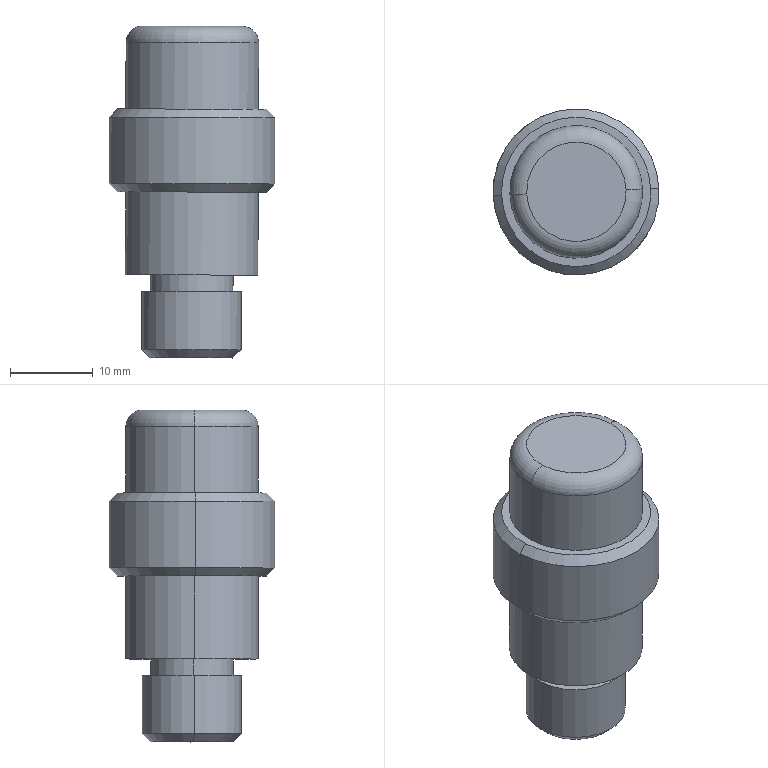Component | SolidWorks | AdjustmentKnob-1 | 1 solid | 24 faces | box 20.03 x 20 x 40.03 mm | volume 8105 mm3 | cylinder 10 | cone 6 | plane 6 | torus 2 | commonest cylinder face diameters 16 x4 12 x2 10 x2 20 x2
build123d program:
from build123d import *

# Parameters (mm, degrees)
FILLET1_R     = 2
CHAMFER1_SIZE = 1


with BuildPart() as part:
    # Sketch1 → Revolve1 (revolve)
    with BuildSketch(Plane.XY, mode=Mode.PRIVATE) as revolve1_sk:
        Polygon((0, 0), (0, 8), (10, 8), (10, 10), (20, 10), (20, 8), (30, 8), (30, 5), (32, 5), (32, 6), (40, 6), (40, 0), align=None)
    revolve(revolve1_sk.sketch.rotate(Axis((0, 0, 0), (1, 0, 0)), 90), axis=Axis((0, 0, 0), (1, 0, 0)))

    # Fillet1
    fillet1_edges = [part.edges().sort_by_distance(p)[0] for p in [
        (0, 0, -8),
    ]]
    fillet(fillet1_edges, radius=FILLET1_R)

    # Chamfer1
    chamfer1_edges = [part.edges().sort_by_distance(p)[0] for p in [
        (20, 0, -10),
        (10, 0, -10),
        (40, 0, -6),
    ]]
    chamfer(chamfer1_edges, length=CHAMFER1_SIZE)


solid = part.part

# Placed as in the assembly
solid = solid.moved(Location((-15.28, 70.983, 1052.851), (90.062, 19.152, -90.191)))
STEP:
#1=COLOUR_RGB('',0.7922,0.8196,0.9333);
#2=FILL_AREA_STYLE_COLOUR('',#1);
#3=FILL_AREA_STYLE('',(#2));
#4=SURFACE_STYLE_FILL_AREA(#3);
#5=SURFACE_SIDE_STYLE('',(#4));
#6=SURFACE_STYLE_USAGE(.BOTH.,#5);
#7=PRESENTATION_STYLE_ASSIGNMENT((#6));
#8=CARTESIAN_POINT('',(-0.9568,2.779,41.058));
#9=VERTEX_POINT('',#8);
#10=CARTESIAN_POINT('',(-0.2488,2.81,41.056));
#11=VERTEX_POINT('',#10);
#12=CARTESIAN_POINT('',(-0.6028,2.795,41.057));
#13=DIRECTION('',(0.003141,0.,1.));
#14=DIRECTION('',(0.9991,0.04346,-0.003138));
#15=AXIS2_PLACEMENT_3D('',#12,#13,#14);
#16=CIRCLE('',#15,0.3543);
#17=EDGE_CURVE('',#9,#11,#16,.T.);
#18=ORIENTED_EDGE('',*,*,#17,.F.);
#19=CARTESIAN_POINT('',(-0.9963,2.777,41.019));
#20=VERTEX_POINT('',#19);
#21=CARTESIAN_POINT('',(-0.9568,2.779,41.058));
#22=DIRECTION('',(-0.7087,-0.03073,-0.7049));
#23=VECTOR('',#22,39.37);
#24=LINE('',#21,#23);
#25=EDGE_CURVE('',#9,#20,#24,.T.);
#26=ORIENTED_EDGE('',*,*,#25,.T.);
#27=CARTESIAN_POINT('',(-0.2096,2.812,41.017));
#28=VERTEX_POINT('',#27);
#29=CARTESIAN_POINT('',(-0.6029,2.795,41.018));
#30=DIRECTION('',(-0.003141,-0.,-1.));
#31=DIRECTION('',(0.9991,0.04346,-0.003138));
#32=AXIS2_PLACEMENT_3D('',#29,#30,#31);
#33=CIRCLE('',#32,0.3937);
#34=EDGE_CURVE('',#28,#20,#33,.T.);
#35=ORIENTED_EDGE('',*,*,#34,.F.);
#36=CARTESIAN_POINT('',(-0.2488,2.81,41.056));
#37=DIRECTION('',(0.7042,0.03073,-0.7093));
#38=VECTOR('',#37,39.37);
#39=LINE('',#36,#38);
#40=EDGE_CURVE('',#11,#28,#39,.T.);
#41=ORIENTED_EDGE('',*,*,#40,.F.);
#42=EDGE_LOOP('',(#18,#26,#35,#41));
#43=FACE_OUTER_BOUND('',#42,.T.);
#44=CARTESIAN_POINT('',(-0.6028,2.795,41.057));
#45=DIRECTION('',(-0.003141,-0.,-1.));
#46=DIRECTION('',(0.9991,0.04346,-0.003138));
#47=AXIS2_PLACEMENT_3D('',#44,#45,#46);
#48=CONICAL_SURFACE('',#47,0.3543,0.7854);
#49=ADVANCED_FACE('',(#43),#48,.T.);
#50=CARTESIAN_POINT('',(-0.25,2.81,40.662));
#51=VERTEX_POINT('',#50);
#52=CARTESIAN_POINT('',(-0.958,2.779,40.665));
#53=VERTEX_POINT('',#52);
#54=CARTESIAN_POINT('',(-0.604,2.795,40.663));
#55=DIRECTION('',(-0.003141,-0.,-1.));
#56=DIRECTION('',(-0.9991,-0.04346,0.003138));
#57=AXIS2_PLACEMENT_3D('',#54,#55,#56);
#58=CIRCLE('',#57,0.3543);
#59=EDGE_CURVE('',#51,#53,#58,.T.);
#60=ORIENTED_EDGE('',*,*,#59,.F.);
#61=CARTESIAN_POINT('',(-0.2106,2.812,40.702));
#62=VERTEX_POINT('',#61);
#63=CARTESIAN_POINT('',(-0.2106,2.812,40.702));
#64=DIRECTION('',(0.7087,0.03073,0.7049));
#65=VECTOR('',#64,39.37);
#66=LINE('',#63,#65);
#67=EDGE_CURVE('',#51,#62,#66,.T.);
#68=ORIENTED_EDGE('',*,*,#67,.T.);
#69=CARTESIAN_POINT('',(-0.9972,2.777,40.704));
#70=VERTEX_POINT('',#69);
#71=CARTESIAN_POINT('',(-0.6039,2.795,40.703));
#72=DIRECTION('',(0.003141,0.,1.));
#73=DIRECTION('',(-0.9991,-0.04346,0.003138));
#74=AXIS2_PLACEMENT_3D('',#71,#72,#73);
#75=CIRCLE('',#74,0.3937);
#76=EDGE_CURVE('',#70,#62,#75,.T.);
#77=ORIENTED_EDGE('',*,*,#76,.F.);
#78=CARTESIAN_POINT('',(-0.9972,2.777,40.704));
#79=DIRECTION('',(-0.7042,-0.03073,0.7093));
#80=VECTOR('',#79,39.37);
#81=LINE('',#78,#80);
#82=EDGE_CURVE('',#53,#70,#81,.T.);
#83=ORIENTED_EDGE('',*,*,#82,.F.);
#84=EDGE_LOOP('',(#60,#68,#77,#83));
#85=FACE_OUTER_BOUND('',#84,.T.);
#86=CARTESIAN_POINT('',(-0.6039,2.795,40.703));
#87=DIRECTION('',(0.003141,0.,1.));
#88=DIRECTION('',(-0.9991,-0.04346,0.003138));
#89=AXIS2_PLACEMENT_3D('',#86,#87,#88);
#90=CONICAL_SURFACE('',#89,0.3937,0.7854);
#91=ADVANCED_FACE('',(#85),#90,.T.);
#92=CARTESIAN_POINT('',(-0.4098,2.803,39.875));
#93=VERTEX_POINT('',#92);
#94=CARTESIAN_POINT('',(-0.8032,2.786,39.877));
#95=VERTEX_POINT('',#94);
#96=CARTESIAN_POINT('',(-0.6065,2.795,39.876));
#97=DIRECTION('',(-0.003141,-0.,-1.));
#98=DIRECTION('',(-0.9991,-0.04346,0.003138));
#99=AXIS2_PLACEMENT_3D('',#96,#97,#98);
#100=CIRCLE('',#99,0.1969);
#101=EDGE_CURVE('',#93,#95,#100,.T.);
#102=ORIENTED_EDGE('',*,*,#101,.F.);
#103=CARTESIAN_POINT('',(-0.3704,2.805,39.915));
#104=VERTEX_POINT('',#103);
#105=CARTESIAN_POINT('',(-0.3704,2.805,39.915));
#106=DIRECTION('',(0.7087,0.03073,0.7049));
#107=VECTOR('',#106,39.37);
#108=LINE('',#105,#107);
#109=EDGE_CURVE('',#93,#104,#108,.T.);
#110=ORIENTED_EDGE('',*,*,#109,.T.);
#111=CARTESIAN_POINT('',(-0.8424,2.784,39.916));
#112=VERTEX_POINT('',#111);
#113=CARTESIAN_POINT('',(-0.6064,2.795,39.915));
#114=DIRECTION('',(0.003141,0.,1.));
#115=DIRECTION('',(-0.9991,-0.04346,0.003138));
#116=AXIS2_PLACEMENT_3D('',#113,#114,#115);
#117=CIRCLE('',#116,0.2362);
#118=EDGE_CURVE('',#112,#104,#117,.T.);
#119=ORIENTED_EDGE('',*,*,#118,.F.);
#120=CARTESIAN_POINT('',(-0.8424,2.784,39.916));
#121=DIRECTION('',(-0.7042,-0.03073,0.7093));
#122=VECTOR('',#121,39.37);
#123=LINE('',#120,#122);
#124=EDGE_CURVE('',#95,#112,#123,.T.);
#125=ORIENTED_EDGE('',*,*,#124,.F.);
#126=EDGE_LOOP('',(#102,#110,#119,#125));
#127=FACE_OUTER_BOUND('',#126,.T.);
#128=CARTESIAN_POINT('',(-0.6064,2.795,39.915));
#129=DIRECTION('',(0.003141,0.,1.));
#130=DIRECTION('',(-0.9991,-0.04346,0.003138));
#131=AXIS2_PLACEMENT_3D('',#128,#129,#130);
#132=CONICAL_SURFACE('',#131,0.2362,0.7854);
#133=ADVANCED_FACE('',(#127),#132,.T.);
#134=CARTESIAN_POINT('',(-0.8376,2.784,41.452));
#135=VERTEX_POINT('',#134);
#136=CARTESIAN_POINT('',(-0.3656,2.805,41.45));
#137=VERTEX_POINT('',#136);
#138=CARTESIAN_POINT('',(-0.6016,2.795,41.451));
#139=DIRECTION('',(0.003141,0.,1.));
#140=DIRECTION('',(0.9991,0.04346,-0.003138));
#141=AXIS2_PLACEMENT_3D('',#138,#139,#140);
#142=CIRCLE('',#141,0.2362);
#143=EDGE_CURVE('',#135,#137,#142,.T.);
#144=ORIENTED_EDGE('',*,*,#143,.F.);
#145=CARTESIAN_POINT('',(-0.9165,2.781,41.373));
#146=VERTEX_POINT('',#145);
#147=CARTESIAN_POINT('',(-0.8378,2.784,41.373));
#148=DIRECTION('',(0.04346,-0.9991,-0.0001365));
#149=DIRECTION('',(0.9991,0.04346,0.));
#150=AXIS2_PLACEMENT_3D('',#147,#148,#149);
#151=CIRCLE('',#150,0.07874);
#152=EDGE_CURVE('',#135,#146,#151,.T.);
#153=ORIENTED_EDGE('',*,*,#152,.T.);
#154=CARTESIAN_POINT('',(-0.2872,2.808,41.371));
#155=VERTEX_POINT('',#154);
#156=CARTESIAN_POINT('',(-0.6018,2.795,41.372));
#157=DIRECTION('',(-0.003141,-0.,-1.));
#158=DIRECTION('',(0.9991,0.04346,-0.003138));
#159=AXIS2_PLACEMENT_3D('',#156,#157,#158);
#160=CIRCLE('',#159,0.315);
#161=EDGE_CURVE('',#155,#146,#160,.T.);
#162=ORIENTED_EDGE('',*,*,#161,.F.);
#163=CARTESIAN_POINT('',(-0.3658,2.805,41.371));
#164=DIRECTION('',(-0.04346,0.9991,0.0001365));
#165=DIRECTION('',(-0.9991,-0.04346,0.));
#166=AXIS2_PLACEMENT_3D('',#163,#164,#165);
#167=CIRCLE('',#166,0.07874);
#168=EDGE_CURVE('',#137,#155,#167,.T.);
#169=ORIENTED_EDGE('',*,*,#168,.F.);
#170=EDGE_LOOP('',(#144,#153,#162,#169));
#171=FACE_OUTER_BOUND('',#170,.T.);
#172=CARTESIAN_POINT('',(-0.6018,2.795,41.372));
#173=DIRECTION('',(-0.003141,-0.,-1.));
#174=DIRECTION('',(0.9991,0.04346,-0.003138));
#175=AXIS2_PLACEMENT_3D('',#172,#173,#174);
#176=TOROIDAL_SURFACE('',#175,0.2362,0.07874);
#177=ADVANCED_FACE('',(#171),#176,.T.);
#178=ORIENTED_EDGE('',*,*,#118,.T.);
#179=CARTESIAN_POINT('',(-0.3695,2.805,40.19));
#180=VERTEX_POINT('',#179);
#181=CARTESIAN_POINT('',(-0.3656,2.805,41.45));
#182=DIRECTION('',(0.003141,0.,1.));
#183=VECTOR('',#182,39.37);
#184=LINE('',#181,#183);
#185=EDGE_CURVE('',#104,#180,#184,.T.);
#186=ORIENTED_EDGE('',*,*,#185,.T.);
#187=CARTESIAN_POINT('',(-0.8415,2.784,40.192));
#188=VERTEX_POINT('',#187);
#189=CARTESIAN_POINT('',(-0.6055,2.795,40.191));
#190=DIRECTION('',(0.003141,0.,1.));
#191=DIRECTION('',(-0.9991,-0.04346,0.003138));
#192=AXIS2_PLACEMENT_3D('',#189,#190,#191);
#193=CIRCLE('',#192,0.2362);
#194=EDGE_CURVE('',#188,#180,#193,.T.);
#195=ORIENTED_EDGE('',*,*,#194,.F.);
#196=CARTESIAN_POINT('',(-0.8376,2.784,41.452));
#197=DIRECTION('',(0.003141,0.,1.));
#198=VECTOR('',#197,39.37);
#199=LINE('',#196,#198);
#200=EDGE_CURVE('',#112,#188,#199,.T.);
#201=ORIENTED_EDGE('',*,*,#200,.F.);
#202=EDGE_LOOP('',(#178,#186,#195,#201));
#203=FACE_OUTER_BOUND('',#202,.T.);
#204=CARTESIAN_POINT('',(-0.6016,2.795,41.451));
#205=DIRECTION('',(0.003141,0.,1.));
#206=DIRECTION('',(-0.9991,-0.04346,0.003138));
#207=AXIS2_PLACEMENT_3D('',#204,#205,#206);
#208=CYLINDRICAL_SURFACE('',#207,0.2362);
#209=ADVANCED_FACE('',(#203),#208,.T.);
#210=CARTESIAN_POINT('',(-0.8022,2.786,40.192));
#211=VERTEX_POINT('',#210);
#212=CARTESIAN_POINT('',(-0.4089,2.803,40.19));
#213=VERTEX_POINT('',#212);
#214=CARTESIAN_POINT('',(-0.6055,2.795,40.191));
#215=DIRECTION('',(0.003141,0.,1.));
#216=DIRECTION('',(-0.9991,-0.04346,0.003138));
#217=AXIS2_PLACEMENT_3D('',#214,#215,#216);
#218=CIRCLE('',#217,0.1969);
#219=EDGE_CURVE('',#211,#213,#218,.T.);
#220=ORIENTED_EDGE('',*,*,#219,.T.);
#221=CARTESIAN_POINT('',(-0.4086,2.803,40.269));
#222=VERTEX_POINT('',#221);
#223=CARTESIAN_POINT('',(-0.4049,2.803,41.45));
#224=DIRECTION('',(0.003141,0.,1.));
#225=VECTOR('',#224,39.37);
#226=LINE('',#223,#225);
#227=EDGE_CURVE('',#213,#222,#226,.T.);
#228=ORIENTED_EDGE('',*,*,#227,.T.);
#229=CARTESIAN_POINT('',(-0.8019,2.786,40.27));
#230=VERTEX_POINT('',#229);
#231=CARTESIAN_POINT('',(-0.6053,2.795,40.27));
#232=DIRECTION('',(0.003141,0.,1.));
#233=DIRECTION('',(-0.9991,-0.04346,0.003138));
#234=AXIS2_PLACEMENT_3D('',#231,#232,#233);
#235=CIRCLE('',#234,0.1969);
#236=EDGE_CURVE('',#230,#222,#235,.T.);
#237=ORIENTED_EDGE('',*,*,#236,.F.);
#238=CARTESIAN_POINT('',(-0.7982,2.786,41.451));
#239=DIRECTION('',(0.003141,0.,1.));
#240=VECTOR('',#239,39.37);
#241=LINE('',#238,#240);
#242=EDGE_CURVE('',#211,#230,#241,.T.);
#243=ORIENTED_EDGE('',*,*,#242,.F.);
#244=EDGE_LOOP('',(#220,#228,#237,#243));
#245=FACE_OUTER_BOUND('',#244,.T.);
#246=CARTESIAN_POINT('',(-0.6016,2.795,41.451));
#247=DIRECTION('',(0.003141,0.,1.));
#248=DIRECTION('',(-0.9991,-0.04346,0.003138));
#249=AXIS2_PLACEMENT_3D('',#246,#247,#248);
#250=CYLINDRICAL_SURFACE('',#249,0.1969);
#251=ADVANCED_FACE('',(#245),#250,.T.);
#252=CARTESIAN_POINT('',(-0.9199,2.781,40.271));
#253=VERTEX_POINT('',#252);
#254=CARTESIAN_POINT('',(-0.2906,2.808,40.269));
#255=VERTEX_POINT('',#254);
#256=CARTESIAN_POINT('',(-0.6053,2.795,40.27));
#257=DIRECTION('',(0.003141,0.,1.));
#258=DIRECTION('',(-0.9991,-0.04346,0.003138));
#259=AXIS2_PLACEMENT_3D('',#256,#257,#258);
#260=CIRCLE('',#259,0.315);
#261=EDGE_CURVE('',#253,#255,#260,.T.);
#262=ORIENTED_EDGE('',*,*,#261,.T.);
#263=CARTESIAN_POINT('',(-0.2894,2.808,40.662));
#264=VERTEX_POINT('',#263);
#265=CARTESIAN_POINT('',(-0.2869,2.808,41.45));
#266=DIRECTION('',(0.003141,0.,1.));
#267=VECTOR('',#266,39.37);
#268=LINE('',#265,#267);
#269=EDGE_CURVE('',#255,#264,#268,.T.);
#270=ORIENTED_EDGE('',*,*,#269,.T.);
#271=CARTESIAN_POINT('',(-0.9187,2.781,40.664));
#272=VERTEX_POINT('',#271);
#273=CARTESIAN_POINT('',(-0.604,2.795,40.663));
#274=DIRECTION('',(0.003141,0.,1.));
#275=DIRECTION('',(-0.9991,-0.04346,0.003138));
#276=AXIS2_PLACEMENT_3D('',#273,#274,#275);
#277=CIRCLE('',#276,0.315);
#278=EDGE_CURVE('',#272,#264,#277,.T.);
#279=ORIENTED_EDGE('',*,*,#278,.F.);
#280=CARTESIAN_POINT('',(-0.9162,2.781,41.452));
#281=DIRECTION('',(0.003141,0.,1.));
#282=VECTOR('',#281,39.37);
#283=LINE('',#280,#282);
#284=EDGE_CURVE('',#253,#272,#283,.T.);
#285=ORIENTED_EDGE('',*,*,#284,.F.);
#286=EDGE_LOOP('',(#262,#270,#279,#285));
#287=FACE_OUTER_BOUND('',#286,.T.);
#288=CARTESIAN_POINT('',(-0.6016,2.795,41.451));
#289=DIRECTION('',(0.003141,0.,1.));
#290=DIRECTION('',(-0.9991,-0.04346,0.003138));
#291=AXIS2_PLACEMENT_3D('',#288,#289,#290);
#292=CYLINDRICAL_SURFACE('',#291,0.315);
#293=ADVANCED_FACE('',(#287),#292,.T.);
#294=ORIENTED_EDGE('',*,*,#76,.T.);
#295=CARTESIAN_POINT('',(-0.2082,2.812,41.45));
#296=DIRECTION('',(0.003141,0.,1.));
#297=VECTOR('',#296,39.37);
#298=LINE('',#295,#297);
#299=EDGE_CURVE('',#62,#28,#298,.T.);
#300=ORIENTED_EDGE('',*,*,#299,.T.);
#301=ORIENTED_EDGE('',*,*,#34,.T.);
#302=CARTESIAN_POINT('',(-0.9949,2.777,41.452));
#303=DIRECTION('',(0.003141,0.,1.));
#304=VECTOR('',#303,39.37);
#305=LINE('',#302,#304);
#306=EDGE_CURVE('',#70,#20,#305,.T.);
#307=ORIENTED_EDGE('',*,*,#306,.F.);
#308=EDGE_LOOP('',(#294,#300,#301,#307));
#309=FACE_OUTER_BOUND('',#308,.T.);
#310=CARTESIAN_POINT('',(-0.6016,2.795,41.451));
#311=DIRECTION('',(0.003141,0.,1.));
#312=DIRECTION('',(-0.9991,-0.04346,0.003138));
#313=AXIS2_PLACEMENT_3D('',#310,#311,#312);
#314=CYLINDRICAL_SURFACE('',#313,0.3937);
#315=ADVANCED_FACE('',(#309),#314,.T.);
#316=CARTESIAN_POINT('',(-0.9175,2.781,41.058));
#317=VERTEX_POINT('',#316);
#318=CARTESIAN_POINT('',(-0.2881,2.808,41.056));
#319=VERTEX_POINT('',#318);
#320=CARTESIAN_POINT('',(-0.6028,2.795,41.057));
#321=DIRECTION('',(0.003141,0.,1.));
#322=DIRECTION('',(-0.9991,-0.04346,0.003138));
#323=AXIS2_PLACEMENT_3D('',#320,#321,#322);
#324=CIRCLE('',#323,0.315);
#325=EDGE_CURVE('',#317,#319,#324,.T.);
#326=ORIENTED_EDGE('',*,*,#325,.T.);
#327=CARTESIAN_POINT('',(-0.2869,2.808,41.45));
#328=DIRECTION('',(0.003141,0.,1.));
#329=VECTOR('',#328,39.37);
#330=LINE('',#327,#329);
#331=EDGE_CURVE('',#319,#155,#330,.T.);
#332=ORIENTED_EDGE('',*,*,#331,.T.);
#333=ORIENTED_EDGE('',*,*,#161,.T.);
#334=CARTESIAN_POINT('',(-0.9162,2.781,41.452));
#335=DIRECTION('',(0.003141,0.,1.));
#336=VECTOR('',#335,39.37);
#337=LINE('',#334,#336);
#338=EDGE_CURVE('',#317,#146,#337,.T.);
#339=ORIENTED_EDGE('',*,*,#338,.F.);
#340=EDGE_LOOP('',(#326,#332,#333,#339));
#341=FACE_OUTER_BOUND('',#340,.T.);
#342=CARTESIAN_POINT('',(-0.6016,2.795,41.451));
#343=DIRECTION('',(0.003141,0.,1.));
#344=DIRECTION('',(-0.9991,-0.04346,0.003138));
#345=AXIS2_PLACEMENT_3D('',#342,#343,#344);
#346=CYLINDRICAL_SURFACE('',#345,0.315);
#347=ADVANCED_FACE('',(#341),#346,.T.);
#348=CARTESIAN_POINT('',(-0.6016,2.795,41.451));
#349=DIRECTION('',(0.003141,0.,1.));
#350=DIRECTION('',(0.9991,0.04346,-0.003138));
#351=AXIS2_PLACEMENT_3D('',#348,#349,#350);
#352=CIRCLE('',#351,0.2362);
#353=EDGE_CURVE('',#137,#135,#352,.T.);
#354=ORIENTED_EDGE('',*,*,#353,.T.);
#355=ORIENTED_EDGE('',*,*,#143,.T.);
#356=EDGE_LOOP('',(#354,#355));
#357=FACE_OUTER_BOUND('',#356,.T.);
#358=CARTESIAN_POINT('',(-0.6016,2.795,41.451));
#359=DIRECTION('',(-0.003141,-0.,-1.));
#360=DIRECTION('',(0.9991,0.04346,-0.003138));
#361=AXIS2_PLACEMENT_3D('',#358,#359,#360);
#362=PLANE('',#361);
#363=ADVANCED_FACE('',(#357),#362,.F.);
#364=ORIENTED_EDGE('',*,*,#331,.F.);
#365=CARTESIAN_POINT('',(-0.6028,2.795,41.057));
#366=DIRECTION('',(0.003141,0.,1.));
#367=DIRECTION('',(-0.9991,-0.04346,0.003138));
#368=AXIS2_PLACEMENT_3D('',#365,#366,#367);
#369=CIRCLE('',#368,0.315);
#370=EDGE_CURVE('',#319,#317,#369,.T.);
#371=ORIENTED_EDGE('',*,*,#370,.T.);
#372=ORIENTED_EDGE('',*,*,#338,.T.);
#373=CARTESIAN_POINT('',(-0.6018,2.795,41.372));
#374=DIRECTION('',(-0.003141,-0.,-1.));
#375=DIRECTION('',(0.9991,0.04346,-0.003138));
#376=AXIS2_PLACEMENT_3D('',#373,#374,#375);
#377=CIRCLE('',#376,0.315);
#378=EDGE_CURVE('',#146,#155,#377,.T.);
#379=ORIENTED_EDGE('',*,*,#378,.T.);
#380=EDGE_LOOP('',(#364,#371,#372,#379));
#381=FACE_OUTER_BOUND('',#380,.T.);
#382=CARTESIAN_POINT('',(-0.6016,2.795,41.451));
#383=DIRECTION('',(0.003141,0.,1.));
#384=DIRECTION('',(-0.9991,-0.04346,0.003138));
#385=AXIS2_PLACEMENT_3D('',#382,#383,#384);
#386=CYLINDRICAL_SURFACE('',#385,0.315);
#387=ADVANCED_FACE('',(#381),#386,.T.);
#388=CARTESIAN_POINT('',(-0.6028,2.795,41.057));
#389=DIRECTION('',(0.003141,0.,1.));
#390=DIRECTION('',(0.9991,0.04346,-0.003138));
#391=AXIS2_PLACEMENT_3D('',#388,#389,#390);
#392=CIRCLE('',#391,0.3543);
#393=EDGE_CURVE('',#11,#9,#392,.T.);
#394=ORIENTED_EDGE('',*,*,#393,.T.);
#395=ORIENTED_EDGE('',*,*,#17,.T.);
#396=EDGE_LOOP('',(#394,#395));
#397=FACE_OUTER_BOUND('',#396,.T.);
#398=ORIENTED_EDGE('',*,*,#325,.F.);
#399=ORIENTED_EDGE('',*,*,#370,.F.);
#400=EDGE_LOOP('',(#398,#399));
#401=FACE_BOUND('',#400,.T.);
#402=CARTESIAN_POINT('',(-0.5891,2.48,41.057));
#403=DIRECTION('',(-0.003141,-0.,-1.));
#404=DIRECTION('',(0.9991,0.04346,-0.003138));
#405=AXIS2_PLACEMENT_3D('',#402,#403,#404);
#406=PLANE('',#405);
#407=ADVANCED_FACE('',(#397,#401),#406,.F.);
#408=ORIENTED_EDGE('',*,*,#299,.F.);
#409=CARTESIAN_POINT('',(-0.6039,2.795,40.703));
#410=DIRECTION('',(0.003141,0.,1.));
#411=DIRECTION('',(-0.9991,-0.04346,0.003138));
#412=AXIS2_PLACEMENT_3D('',#409,#410,#411);
#413=CIRCLE('',#412,0.3937);
#414=EDGE_CURVE('',#62,#70,#413,.T.);
#415=ORIENTED_EDGE('',*,*,#414,.T.);
#416=ORIENTED_EDGE('',*,*,#306,.T.);
#417=CARTESIAN_POINT('',(-0.6029,2.795,41.018));
#418=DIRECTION('',(-0.003141,-0.,-1.));
#419=DIRECTION('',(0.9991,0.04346,-0.003138));
#420=AXIS2_PLACEMENT_3D('',#417,#418,#419);
#421=CIRCLE('',#420,0.3937);
#422=EDGE_CURVE('',#20,#28,#421,.T.);
#423=ORIENTED_EDGE('',*,*,#422,.T.);
#424=EDGE_LOOP('',(#408,#415,#416,#423));
#425=FACE_OUTER_BOUND('',#424,.T.);
#426=CARTESIAN_POINT('',(-0.6016,2.795,41.451));
#427=DIRECTION('',(0.003141,0.,1.));
#428=DIRECTION('',(-0.9991,-0.04346,0.003138));
#429=AXIS2_PLACEMENT_3D('',#426,#427,#428);
#430=CYLINDRICAL_SURFACE('',#429,0.3937);
#431=ADVANCED_FACE('',(#425),#430,.T.);
#432=CARTESIAN_POINT('',(-0.604,2.795,40.663));
#433=DIRECTION('',(-0.003141,-0.,-1.));
#434=DIRECTION('',(-0.9991,-0.04346,0.003138));
#435=AXIS2_PLACEMENT_3D('',#432,#433,#434);
#436=CIRCLE('',#435,0.3543);
#437=EDGE_CURVE('',#53,#51,#436,.T.);
#438=ORIENTED_EDGE('',*,*,#437,.T.);
#439=ORIENTED_EDGE('',*,*,#59,.T.);
#440=EDGE_LOOP('',(#438,#439));
#441=FACE_OUTER_BOUND('',#440,.T.);
#442=ORIENTED_EDGE('',*,*,#278,.T.);
#443=CARTESIAN_POINT('',(-0.604,2.795,40.663));
#444=DIRECTION('',(0.003141,0.,1.));
#445=DIRECTION('',(-0.9991,-0.04346,0.003138));
#446=AXIS2_PLACEMENT_3D('',#443,#444,#445);
#447=CIRCLE('',#446,0.315);
#448=EDGE_CURVE('',#264,#272,#447,.T.);
#449=ORIENTED_EDGE('',*,*,#448,.T.);
#450=EDGE_LOOP('',(#442,#449));
#451=FACE_BOUND('',#450,.T.);
#452=CARTESIAN_POINT('',(-0.5869,2.401,40.663));
#453=DIRECTION('',(0.003141,0.,1.));
#454=DIRECTION('',(-0.9991,-0.04346,0.003138));
#455=AXIS2_PLACEMENT_3D('',#452,#453,#454);
#456=PLANE('',#455);
#457=ADVANCED_FACE('',(#441,#451),#456,.F.);
#458=ORIENTED_EDGE('',*,*,#269,.F.);
#459=CARTESIAN_POINT('',(-0.6053,2.795,40.27));
#460=DIRECTION('',(0.003141,0.,1.));
#461=DIRECTION('',(-0.9991,-0.04346,0.003138));
#462=AXIS2_PLACEMENT_3D('',#459,#460,#461);
#463=CIRCLE('',#462,0.315);
#464=EDGE_CURVE('',#255,#253,#463,.T.);
#465=ORIENTED_EDGE('',*,*,#464,.T.);
#466=ORIENTED_EDGE('',*,*,#284,.T.);
#467=ORIENTED_EDGE('',*,*,#448,.F.);
#468=EDGE_LOOP('',(#458,#465,#466,#467));
#469=FACE_OUTER_BOUND('',#468,.T.);
#470=CARTESIAN_POINT('',(-0.6016,2.795,41.451));
#471=DIRECTION('',(0.003141,0.,1.));
#472=DIRECTION('',(-0.9991,-0.04346,0.003138));
#473=AXIS2_PLACEMENT_3D('',#470,#471,#472);
#474=CYLINDRICAL_SURFACE('',#473,0.315);
#475=ADVANCED_FACE('',(#469),#474,.T.);
#476=ORIENTED_EDGE('',*,*,#261,.F.);
#477=ORIENTED_EDGE('',*,*,#464,.F.);
#478=EDGE_LOOP('',(#476,#477));
#479=FACE_OUTER_BOUND('',#478,.T.);
#480=ORIENTED_EDGE('',*,*,#236,.T.);
#481=CARTESIAN_POINT('',(-0.6053,2.795,40.27));
#482=DIRECTION('',(0.003141,0.,1.));
#483=DIRECTION('',(-0.9991,-0.04346,0.003138));
#484=AXIS2_PLACEMENT_3D('',#481,#482,#483);
#485=CIRCLE('',#484,0.1969);
#486=EDGE_CURVE('',#222,#230,#485,.T.);
#487=ORIENTED_EDGE('',*,*,#486,.T.);
#488=EDGE_LOOP('',(#480,#487));
#489=FACE_BOUND('',#488,.T.);
#490=CARTESIAN_POINT('',(-0.5916,2.48,40.27));
#491=DIRECTION('',(0.003141,0.,1.));
#492=DIRECTION('',(-0.9991,-0.04346,0.003138));
#493=AXIS2_PLACEMENT_3D('',#490,#491,#492);
#494=PLANE('',#493);
#495=ADVANCED_FACE('',(#479,#489),#494,.F.);
#496=ORIENTED_EDGE('',*,*,#227,.F.);
#497=CARTESIAN_POINT('',(-0.6055,2.795,40.191));
#498=DIRECTION('',(0.003141,0.,1.));
#499=DIRECTION('',(-0.9991,-0.04346,0.003138));
#500=AXIS2_PLACEMENT_3D('',#497,#498,#499);
#501=CIRCLE('',#500,0.1969);
#502=EDGE_CURVE('',#213,#211,#501,.T.);
#503=ORIENTED_EDGE('',*,*,#502,.T.);
#504=ORIENTED_EDGE('',*,*,#242,.T.);
#505=ORIENTED_EDGE('',*,*,#486,.F.);
#506=EDGE_LOOP('',(#496,#503,#504,#505));
#507=FACE_OUTER_BOUND('',#506,.T.);
#508=CARTESIAN_POINT('',(-0.6016,2.795,41.451));
#509=DIRECTION('',(0.003141,0.,1.));
#510=DIRECTION('',(-0.9991,-0.04346,0.003138));
#511=AXIS2_PLACEMENT_3D('',#508,#509,#510);
#512=CYLINDRICAL_SURFACE('',#511,0.1969);
#513=ADVANCED_FACE('',(#507),#512,.T.);
#514=ORIENTED_EDGE('',*,*,#219,.F.);
#515=ORIENTED_EDGE('',*,*,#502,.F.);
#516=EDGE_LOOP('',(#514,#515));
#517=FACE_BOUND('',#516,.T.);
#518=ORIENTED_EDGE('',*,*,#194,.T.);
#519=CARTESIAN_POINT('',(-0.6055,2.795,40.191));
#520=DIRECTION('',(0.003141,0.,1.));
#521=DIRECTION('',(-0.9991,-0.04346,0.003138));
#522=AXIS2_PLACEMENT_3D('',#519,#520,#521);
#523=CIRCLE('',#522,0.2362);
#524=EDGE_CURVE('',#180,#188,#523,.T.);
#525=ORIENTED_EDGE('',*,*,#524,.T.);
#526=EDGE_LOOP('',(#518,#525));
#527=FACE_OUTER_BOUND('',#526,.T.);
#528=CARTESIAN_POINT('',(-0.597,2.598,40.191));
#529=DIRECTION('',(-0.003141,-0.,-1.));
#530=DIRECTION('',(0.9991,0.04346,-0.003138));
#531=AXIS2_PLACEMENT_3D('',#528,#529,#530);
#532=PLANE('',#531);
#533=ADVANCED_FACE('',(#517,#527),#532,.F.);
#534=ORIENTED_EDGE('',*,*,#185,.F.);
#535=CARTESIAN_POINT('',(-0.6064,2.795,39.915));
#536=DIRECTION('',(0.003141,0.,1.));
#537=DIRECTION('',(-0.9991,-0.04346,0.003138));
#538=AXIS2_PLACEMENT_3D('',#535,#536,#537);
#539=CIRCLE('',#538,0.2362);
#540=EDGE_CURVE('',#104,#112,#539,.T.);
#541=ORIENTED_EDGE('',*,*,#540,.T.);
#542=ORIENTED_EDGE('',*,*,#200,.T.);
#543=ORIENTED_EDGE('',*,*,#524,.F.);
#544=EDGE_LOOP('',(#534,#541,#542,#543));
#545=FACE_OUTER_BOUND('',#544,.T.);
#546=CARTESIAN_POINT('',(-0.6016,2.795,41.451));
#547=DIRECTION('',(0.003141,0.,1.));
#548=DIRECTION('',(-0.9991,-0.04346,0.003138));
#549=AXIS2_PLACEMENT_3D('',#546,#547,#548);
#550=CYLINDRICAL_SURFACE('',#549,0.2362);
#551=ADVANCED_FACE('',(#545),#550,.T.);
#552=CARTESIAN_POINT('',(-0.6065,2.795,39.876));
#553=DIRECTION('',(-0.003141,-0.,-1.));
#554=DIRECTION('',(-0.9991,-0.04346,0.003138));
#555=AXIS2_PLACEMENT_3D('',#552,#553,#554);
#556=CIRCLE('',#555,0.1969);
#557=EDGE_CURVE('',#95,#93,#556,.T.);
#558=ORIENTED_EDGE('',*,*,#557,.T.);
#559=ORIENTED_EDGE('',*,*,#101,.T.);
#560=EDGE_LOOP('',(#558,#559));
#561=FACE_OUTER_BOUND('',#560,.T.);
#562=CARTESIAN_POINT('',(-0.5962,2.559,39.876));
#563=DIRECTION('',(0.003141,0.,1.));
#564=DIRECTION('',(-0.9991,-0.04346,0.003138));
#565=AXIS2_PLACEMENT_3D('',#562,#563,#564);
#566=PLANE('',#565);
#567=ADVANCED_FACE('',(#561),#566,.F.);
#568=ORIENTED_EDGE('',*,*,#152,.F.);
#569=ORIENTED_EDGE('',*,*,#353,.F.);
#570=ORIENTED_EDGE('',*,*,#168,.T.);
#571=ORIENTED_EDGE('',*,*,#378,.F.);
#572=EDGE_LOOP('',(#568,#569,#570,#571));
#573=FACE_OUTER_BOUND('',#572,.T.);
#574=CARTESIAN_POINT('',(-0.6018,2.795,41.372));
#575=DIRECTION('',(-0.003141,-0.,-1.));
#576=DIRECTION('',(0.9991,0.04346,-0.003138));
#577=AXIS2_PLACEMENT_3D('',#574,#575,#576);
#578=TOROIDAL_SURFACE('',#577,0.2362,0.07874);
#579=ADVANCED_FACE('',(#573),#578,.T.);
#580=ORIENTED_EDGE('',*,*,#109,.F.);
#581=ORIENTED_EDGE('',*,*,#557,.F.);
#582=ORIENTED_EDGE('',*,*,#124,.T.);
#583=ORIENTED_EDGE('',*,*,#540,.F.);
#584=EDGE_LOOP('',(#580,#581,#582,#583));
#585=FACE_OUTER_BOUND('',#584,.T.);
#586=CARTESIAN_POINT('',(-0.6064,2.795,39.915));
#587=DIRECTION('',(0.003141,0.,1.));
#588=DIRECTION('',(-0.9991,-0.04346,0.003138));
#589=AXIS2_PLACEMENT_3D('',#586,#587,#588);
#590=CONICAL_SURFACE('',#589,0.2362,0.7854);
#591=ADVANCED_FACE('',(#585),#590,.T.);
#592=ORIENTED_EDGE('',*,*,#67,.F.);
#593=ORIENTED_EDGE('',*,*,#437,.F.);
#594=ORIENTED_EDGE('',*,*,#82,.T.);
#595=ORIENTED_EDGE('',*,*,#414,.F.);
#596=EDGE_LOOP('',(#592,#593,#594,#595));
#597=FACE_OUTER_BOUND('',#596,.T.);
#598=CARTESIAN_POINT('',(-0.6039,2.795,40.703));
#599=DIRECTION('',(0.003141,0.,1.));
#600=DIRECTION('',(-0.9991,-0.04346,0.003138));
#601=AXIS2_PLACEMENT_3D('',#598,#599,#600);
#602=CONICAL_SURFACE('',#601,0.3937,0.7854);
#603=ADVANCED_FACE('',(#597),#602,.T.);
#604=ORIENTED_EDGE('',*,*,#25,.F.);
#605=ORIENTED_EDGE('',*,*,#393,.F.);
#606=ORIENTED_EDGE('',*,*,#40,.T.);
#607=ORIENTED_EDGE('',*,*,#422,.F.);
#608=EDGE_LOOP('',(#604,#605,#606,#607));
#609=FACE_OUTER_BOUND('',#608,.T.);
#610=CARTESIAN_POINT('',(-0.6028,2.795,41.057));
#611=DIRECTION('',(-0.003141,-0.,-1.));
#612=DIRECTION('',(0.9991,0.04346,-0.003138));
#613=AXIS2_PLACEMENT_3D('',#610,#611,#612);
#614=CONICAL_SURFACE('',#613,0.3543,0.7854);
#615=ADVANCED_FACE('',(#609),#614,.T.);
#616=CLOSED_SHELL('',(#49,#91,#133,#177,#209,#251,#293,#315,#347,#363,#387,#407,#431,#457,#475,#495,#513,#533,#551,#567,#579,#591,#603,#615));
#617=MANIFOLD_SOLID_BREP('',#616);
#618=STYLED_ITEM('',(#7),#617);
#619=(LENGTH_UNIT()NAMED_UNIT(*)SI_UNIT($,.METRE.));
#620=LENGTH_MEASURE_WITH_UNIT(LENGTH_MEASURE(0.0254),#619);
#621=DIMENSIONAL_EXPONENTS(1.,0.,0.,0.,0.,0.,0.);
#622=(CONVERSION_BASED_UNIT('',#620)LENGTH_UNIT()NAMED_UNIT(#621));
#623=UNCERTAINTY_MEASURE_WITH_UNIT(LENGTH_MEASURE(0.00001),#622,'','');
#624=(NAMED_UNIT(*)PLANE_ANGLE_UNIT()SI_UNIT($,.RADIAN.));
#625=(NAMED_UNIT(*)SI_UNIT($,.STERADIAN.)SOLID_ANGLE_UNIT());
#626=(GEOMETRIC_REPRESENTATION_CONTEXT(3)GLOBAL_UNCERTAINTY_ASSIGNED_CONTEXT((#623))GLOBAL_UNIT_ASSIGNED_CONTEXT((#622,#624,#625))REPRESENTATION_CONTEXT('',''));
#627=MECHANICAL_DESIGN_GEOMETRIC_PRESENTATION_REPRESENTATION('',(#618),#626);
#628=PRESENTATION_LAYER_ASSIGNMENT('','',(#618));
#629=CARTESIAN_POINT('',(0.,0.,0.));
#630=DIRECTION('',(0.,0.,1.));
#631=DIRECTION('',(1.,0.,0.));
#632=AXIS2_PLACEMENT_3D('',#629,#630,#631);
#633=(LENGTH_UNIT()NAMED_UNIT(*)SI_UNIT($,.METRE.));
#634=LENGTH_MEASURE_WITH_UNIT(LENGTH_MEASURE(0.0254),#633);
#635=DIMENSIONAL_EXPONENTS(1.,0.,0.,0.,0.,0.,0.);
#636=(CONVERSION_BASED_UNIT('',#634)LENGTH_UNIT()NAMED_UNIT(#635));
#637=UNCERTAINTY_MEASURE_WITH_UNIT(LENGTH_MEASURE(0.00001),#636,'','');
#638=(NAMED_UNIT(*)PLANE_ANGLE_UNIT()SI_UNIT($,.RADIAN.));
#639=(NAMED_UNIT(*)SI_UNIT($,.STERADIAN.)SOLID_ANGLE_UNIT());
#640=(GEOMETRIC_REPRESENTATION_CONTEXT(3)GLOBAL_UNCERTAINTY_ASSIGNED_CONTEXT((#637))GLOBAL_UNIT_ASSIGNED_CONTEXT((#636,#638,#639))REPRESENTATION_CONTEXT('',''));
#641=ADVANCED_BREP_SHAPE_REPRESENTATION('',(#617,#632),#640);